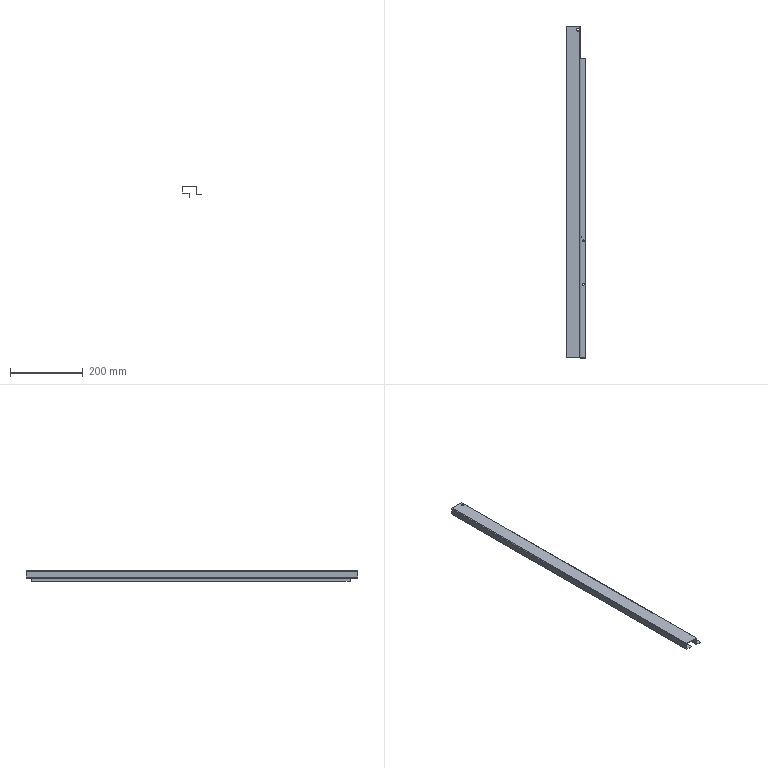Component | SolidWorks | CCQ-1.1-16LowerSidePost3-2 | 1 solid | 60 faces | volume 109153 mm3 | plane 44 | cylinder 16 | commonest cylinder face diameters 1.473 x5 3.473 x5 5 x4 8 x2 | material 304